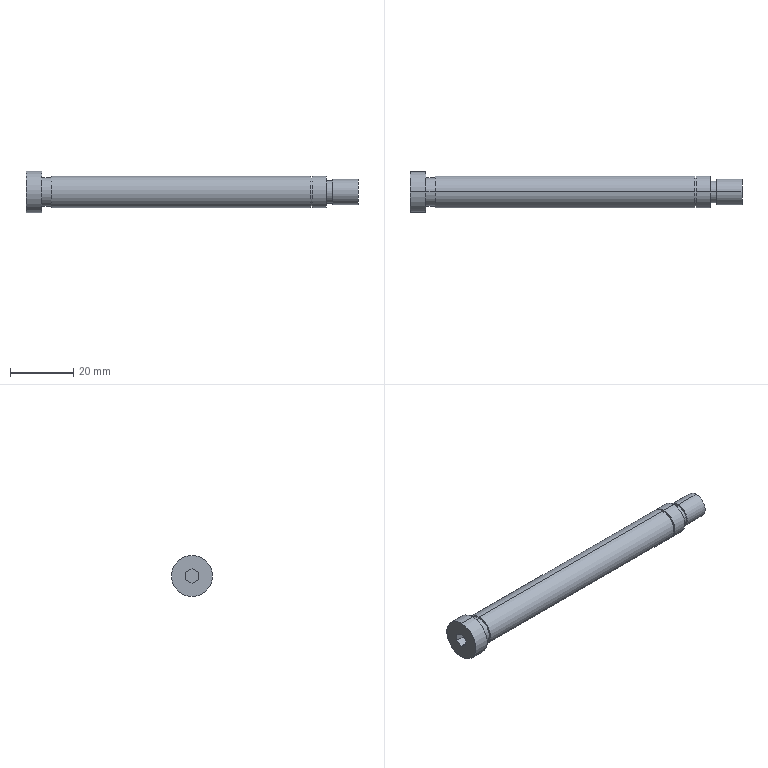Component | SolidWorks | ElectricalBoxAssembly2-1_M8-10-16-90GuidePinBolt-1 | 1 solid | 29 faces | box 105 x 13 x 13 mm | volume 8090 mm3 | plane 15 | cylinder 14 | commonest cylinder face diameters 10 x4 9 x4 7 x2 8 x2 13 x2
build123d program:
from build123d import *

# Parameters (mm, degrees)
SKETCH1_R           = 6.5
BOSS_EXTRUDE1_DEPTH = 5
SKETCH2_R           = 5
BOSS_EXTRUDE2_DEPTH = 90
SKETCH3_R           = 4
BOSS_EXTRUDE3_DEPTH = 10
SKETCH4_R           = 5
SKETCH4_R_2         = 4.5
CUT_EXTRUDE1_DEPTH  = 3
SKETCH5_R           = 4
SKETCH5_R_2         = 3.5
CUT_EXTRUDE2_DEPTH  = 2
CUT_EXTRUDE3_DEPTH  = 5
SKETCH7_W           = 0.5
SKETCH7_H           = 1


with BuildPart() as part:
    # Sketch1 → Boss-Extrude1 (new body)
    with BuildSketch(Plane.XY):
        Circle(SKETCH1_R)
    extrude(amount=-BOSS_EXTRUDE1_DEPTH)

    # Sketch2 → Boss-Extrude2 (add)
    with BuildSketch(Plane(origin=(0, 0, -5), x_dir=(-1, 0, 0), z_dir=(0, 0, -1))):
        with Locations(Location((0, 0, 0), (0, 0, 180))):
            Circle(SKETCH2_R)
    extrude(amount=BOSS_EXTRUDE2_DEPTH)

    # Sketch3 → Boss-Extrude3 (add)
    with BuildSketch(Plane(origin=(0, 0, -95), x_dir=(-1, 0, 0), z_dir=(0, 0, -1))):
        Circle(SKETCH3_R)
    extrude(amount=BOSS_EXTRUDE3_DEPTH)

    # Sketch4 → Cut-Extrude1 (cut)
    with BuildSketch(Plane(origin=(0, 0, -5), x_dir=(-1, 0, 0), z_dir=(0, 0, -1))):
        with Locations(Location((0, 0, 0), (0, 0, 180))):
            Circle(SKETCH4_R)
        Circle(SKETCH4_R_2, mode=Mode.SUBTRACT)
    extrude(amount=CUT_EXTRUDE1_DEPTH, mode=Mode.SUBTRACT)

    # Sketch5 → Cut-Extrude2 (cut)
    with BuildSketch(Plane(origin=(0, 0, -95), x_dir=(-1, 0, 0), z_dir=(0, 0, -1))):
        Circle(SKETCH5_R)
        Circle(SKETCH5_R_2, mode=Mode.SUBTRACT)
    extrude(amount=CUT_EXTRUDE2_DEPTH, mode=Mode.SUBTRACT)

    # Sketch6 → Cut-Extrude3 (cut)
    with BuildSketch(Plane.XY):
        Polygon((2.309, 0), (1.155, 2), (-1.155, 2), (-2.309, 0), (-1.155, -2), (1.155, -2), align=None)
    extrude(amount=-CUT_EXTRUDE3_DEPTH, mode=Mode.SUBTRACT)

    # Sketch7 → Cut-Revolve1 (revolve, cut)
    with BuildSketch(Plane(origin=(0, 0, 0), x_dir=(0, 0, -1), z_dir=(1, 0, 0)), mode=Mode.PRIVATE) as cut_revolve1_sk:
        with Locations((90.25, 5)):
            Rectangle(SKETCH7_W, SKETCH7_H)
    revolve(cut_revolve1_sk.sketch.rotate(Axis((0, 0, 0), (0, 0, -1)), 90), axis=Axis((0, 0, 0), (0, 0, -1)), mode=Mode.SUBTRACT)


solid = part.part

# Placed as in the assembly
solid = solid.moved(Location((640.968, 334.666, 1526.399), (0, -90, 0)))
STEP:
#1=COLOUR_RGB('',0.7922,0.8196,0.9333);
#2=FILL_AREA_STYLE_COLOUR('',#1);
#3=FILL_AREA_STYLE('',(#2));
#4=SURFACE_STYLE_FILL_AREA(#3);
#5=SURFACE_SIDE_STYLE('',(#4));
#6=SURFACE_STYLE_USAGE(.BOTH.,#5);
#7=PRESENTATION_STYLE_ASSIGNMENT((#6));
#8=CARTESIAN_POINT('',(28.975,13.176,60.291));
#9=VERTEX_POINT('',#8);
#10=CARTESIAN_POINT('',(28.975,13.176,59.898));
#11=VERTEX_POINT('',#10);
#12=CARTESIAN_POINT('',(28.975,13.176,60.094));
#13=DIRECTION('',(1.,0.,0.));
#14=DIRECTION('',(0.,0.,1.));
#15=AXIS2_PLACEMENT_3D('',#12,#13,#14);
#16=CIRCLE('',#15,0.1969);
#17=EDGE_CURVE('',#9,#11,#16,.T.);
#18=ORIENTED_EDGE('',*,*,#17,.F.);
#19=CARTESIAN_POINT('',(28.798,13.176,60.291));
#20=VERTEX_POINT('',#19);
#21=CARTESIAN_POINT('',(28.975,13.176,60.291));
#22=DIRECTION('',(-1.,-0.,-0.));
#23=VECTOR('',#22,39.37);
#24=LINE('',#21,#23);
#25=EDGE_CURVE('',#9,#20,#24,.T.);
#26=ORIENTED_EDGE('',*,*,#25,.T.);
#27=CARTESIAN_POINT('',(28.798,13.176,59.898));
#28=VERTEX_POINT('',#27);
#29=CARTESIAN_POINT('',(28.798,13.176,60.094));
#30=DIRECTION('',(-1.,-0.,-0.));
#31=DIRECTION('',(0.,1.,0.));
#32=AXIS2_PLACEMENT_3D('',#29,#30,#31);
#33=CIRCLE('',#32,0.1969);
#34=EDGE_CURVE('',#28,#20,#33,.T.);
#35=ORIENTED_EDGE('',*,*,#34,.F.);
#36=CARTESIAN_POINT('',(28.975,13.176,59.898));
#37=DIRECTION('',(-1.,-0.,-0.));
#38=VECTOR('',#37,39.37);
#39=LINE('',#36,#38);
#40=EDGE_CURVE('',#11,#28,#39,.T.);
#41=ORIENTED_EDGE('',*,*,#40,.F.);
#42=EDGE_LOOP('',(#18,#26,#35,#41));
#43=FACE_OUTER_BOUND('',#42,.T.);
#44=CARTESIAN_POINT('',(28.975,13.176,60.094));
#45=DIRECTION('',(-1.,-0.,-0.));
#46=DIRECTION('',(0.,0.,-1.));
#47=AXIS2_PLACEMENT_3D('',#44,#45,#46);
#48=CYLINDRICAL_SURFACE('',#47,0.1969);
#49=ADVANCED_FACE('',(#43),#48,.T.);
#50=CARTESIAN_POINT('',(29.054,13.176,60.232));
#51=VERTEX_POINT('',#50);
#52=CARTESIAN_POINT('',(29.054,13.176,59.957));
#53=VERTEX_POINT('',#52);
#54=CARTESIAN_POINT('',(29.054,13.176,60.094));
#55=DIRECTION('',(1.,0.,0.));
#56=DIRECTION('',(0.,0.,1.));
#57=AXIS2_PLACEMENT_3D('',#54,#55,#56);
#58=CIRCLE('',#57,0.1378);
#59=EDGE_CURVE('',#51,#53,#58,.T.);
#60=ORIENTED_EDGE('',*,*,#59,.F.);
#61=CARTESIAN_POINT('',(28.975,13.176,60.232));
#62=VERTEX_POINT('',#61);
#63=CARTESIAN_POINT('',(29.054,13.176,60.232));
#64=DIRECTION('',(-1.,-0.,-0.));
#65=VECTOR('',#64,39.37);
#66=LINE('',#63,#65);
#67=EDGE_CURVE('',#51,#62,#66,.T.);
#68=ORIENTED_EDGE('',*,*,#67,.T.);
#69=CARTESIAN_POINT('',(28.975,13.176,59.957));
#70=VERTEX_POINT('',#69);
#71=CARTESIAN_POINT('',(28.975,13.176,60.094));
#72=DIRECTION('',(1.,0.,0.));
#73=DIRECTION('',(0.,0.,1.));
#74=AXIS2_PLACEMENT_3D('',#71,#72,#73);
#75=CIRCLE('',#74,0.1378);
#76=EDGE_CURVE('',#62,#70,#75,.T.);
#77=ORIENTED_EDGE('',*,*,#76,.T.);
#78=CARTESIAN_POINT('',(29.054,13.176,59.957));
#79=DIRECTION('',(-1.,-0.,-0.));
#80=VECTOR('',#79,39.37);
#81=LINE('',#78,#80);
#82=EDGE_CURVE('',#53,#70,#81,.T.);
#83=ORIENTED_EDGE('',*,*,#82,.F.);
#84=EDGE_LOOP('',(#60,#68,#77,#83));
#85=FACE_OUTER_BOUND('',#84,.T.);
#86=CARTESIAN_POINT('',(29.054,13.176,60.094));
#87=DIRECTION('',(-1.,-0.,-0.));
#88=DIRECTION('',(0.,0.,-1.));
#89=AXIS2_PLACEMENT_3D('',#86,#87,#88);
#90=CYLINDRICAL_SURFACE('',#89,0.1378);
#91=ADVANCED_FACE('',(#85),#90,.T.);
#92=CARTESIAN_POINT('',(29.369,13.176,60.252));
#93=VERTEX_POINT('',#92);
#94=CARTESIAN_POINT('',(29.369,13.176,59.937));
#95=VERTEX_POINT('',#94);
#96=CARTESIAN_POINT('',(29.369,13.176,60.094));
#97=DIRECTION('',(1.,0.,0.));
#98=DIRECTION('',(0.,0.,1.));
#99=AXIS2_PLACEMENT_3D('',#96,#97,#98);
#100=CIRCLE('',#99,0.1575);
#101=EDGE_CURVE('',#93,#95,#100,.T.);
#102=ORIENTED_EDGE('',*,*,#101,.F.);
#103=CARTESIAN_POINT('',(29.054,13.176,60.252));
#104=VERTEX_POINT('',#103);
#105=CARTESIAN_POINT('',(29.369,13.176,60.252));
#106=DIRECTION('',(-1.,-0.,-0.));
#107=VECTOR('',#106,39.37);
#108=LINE('',#105,#107);
#109=EDGE_CURVE('',#93,#104,#108,.T.);
#110=ORIENTED_EDGE('',*,*,#109,.T.);
#111=CARTESIAN_POINT('',(29.054,13.176,59.937));
#112=VERTEX_POINT('',#111);
#113=CARTESIAN_POINT('',(29.054,13.176,60.094));
#114=DIRECTION('',(1.,0.,0.));
#115=DIRECTION('',(0.,0.,1.));
#116=AXIS2_PLACEMENT_3D('',#113,#114,#115);
#117=CIRCLE('',#116,0.1575);
#118=EDGE_CURVE('',#104,#112,#117,.T.);
#119=ORIENTED_EDGE('',*,*,#118,.T.);
#120=CARTESIAN_POINT('',(29.369,13.176,59.937));
#121=DIRECTION('',(-1.,-0.,-0.));
#122=VECTOR('',#121,39.37);
#123=LINE('',#120,#122);
#124=EDGE_CURVE('',#95,#112,#123,.T.);
#125=ORIENTED_EDGE('',*,*,#124,.F.);
#126=EDGE_LOOP('',(#102,#110,#119,#125));
#127=FACE_OUTER_BOUND('',#126,.T.);
#128=CARTESIAN_POINT('',(29.369,13.176,60.094));
#129=DIRECTION('',(-1.,-0.,-0.));
#130=DIRECTION('',(0.,0.,-1.));
#131=AXIS2_PLACEMENT_3D('',#128,#129,#130);
#132=CYLINDRICAL_SURFACE('',#131,0.1575);
#133=ADVANCED_FACE('',(#127),#132,.T.);
#134=CARTESIAN_POINT('',(28.798,13.353,60.094));
#135=VERTEX_POINT('',#134);
#136=CARTESIAN_POINT('',(28.798,12.999,60.094));
#137=VERTEX_POINT('',#136);
#138=CARTESIAN_POINT('',(28.798,13.176,60.094));
#139=DIRECTION('',(-1.,-0.,-0.));
#140=DIRECTION('',(0.,1.,0.));
#141=AXIS2_PLACEMENT_3D('',#138,#139,#140);
#142=CIRCLE('',#141,0.1772);
#143=EDGE_CURVE('',#135,#137,#142,.T.);
#144=ORIENTED_EDGE('',*,*,#143,.T.);
#145=CARTESIAN_POINT('',(28.778,12.999,60.094));
#146=VERTEX_POINT('',#145);
#147=CARTESIAN_POINT('',(25.235,12.999,60.094));
#148=DIRECTION('',(-1.,-0.,-0.));
#149=VECTOR('',#148,39.37);
#150=LINE('',#147,#149);
#151=EDGE_CURVE('',#137,#146,#150,.T.);
#152=ORIENTED_EDGE('',*,*,#151,.T.);
#153=CARTESIAN_POINT('',(28.778,13.353,60.094));
#154=VERTEX_POINT('',#153);
#155=CARTESIAN_POINT('',(28.778,13.176,60.094));
#156=DIRECTION('',(-1.,-0.,-0.));
#157=DIRECTION('',(0.,1.,0.));
#158=AXIS2_PLACEMENT_3D('',#155,#156,#157);
#159=CIRCLE('',#158,0.1772);
#160=EDGE_CURVE('',#154,#146,#159,.T.);
#161=ORIENTED_EDGE('',*,*,#160,.F.);
#162=CARTESIAN_POINT('',(25.235,13.353,60.094));
#163=DIRECTION('',(-1.,-0.,-0.));
#164=VECTOR('',#163,39.37);
#165=LINE('',#162,#164);
#166=EDGE_CURVE('',#135,#154,#165,.T.);
#167=ORIENTED_EDGE('',*,*,#166,.F.);
#168=EDGE_LOOP('',(#144,#152,#161,#167));
#169=FACE_OUTER_BOUND('',#168,.T.);
#170=CARTESIAN_POINT('',(25.235,13.176,60.094));
#171=DIRECTION('',(-1.,-0.,-0.));
#172=DIRECTION('',(0.,1.,0.));
#173=AXIS2_PLACEMENT_3D('',#170,#171,#172);
#174=CYLINDRICAL_SURFACE('',#173,0.1772);
#175=ADVANCED_FACE('',(#169),#174,.T.);
#176=CARTESIAN_POINT('',(25.432,13.176,59.839));
#177=VERTEX_POINT('',#176);
#178=CARTESIAN_POINT('',(25.432,13.176,60.35));
#179=VERTEX_POINT('',#178);
#180=CARTESIAN_POINT('',(25.432,13.176,60.094));
#181=DIRECTION('',(-1.,-0.,-0.));
#182=DIRECTION('',(0.,0.,-1.));
#183=AXIS2_PLACEMENT_3D('',#180,#181,#182);
#184=CIRCLE('',#183,0.2559);
#185=EDGE_CURVE('',#177,#179,#184,.T.);
#186=ORIENTED_EDGE('',*,*,#185,.T.);
#187=CARTESIAN_POINT('',(25.235,13.176,60.35));
#188=VERTEX_POINT('',#187);
#189=CARTESIAN_POINT('',(25.432,13.176,60.35));
#190=DIRECTION('',(-1.,-0.,-0.));
#191=VECTOR('',#190,39.37);
#192=LINE('',#189,#191);
#193=EDGE_CURVE('',#179,#188,#192,.T.);
#194=ORIENTED_EDGE('',*,*,#193,.T.);
#195=CARTESIAN_POINT('',(25.235,13.176,59.839));
#196=VERTEX_POINT('',#195);
#197=CARTESIAN_POINT('',(25.235,13.176,60.094));
#198=DIRECTION('',(-1.,-0.,-0.));
#199=DIRECTION('',(0.,0.,-1.));
#200=AXIS2_PLACEMENT_3D('',#197,#198,#199);
#201=CIRCLE('',#200,0.2559);
#202=EDGE_CURVE('',#196,#188,#201,.T.);
#203=ORIENTED_EDGE('',*,*,#202,.F.);
#204=CARTESIAN_POINT('',(25.432,13.176,59.839));
#205=DIRECTION('',(-1.,-0.,-0.));
#206=VECTOR('',#205,39.37);
#207=LINE('',#204,#206);
#208=EDGE_CURVE('',#177,#196,#207,.T.);
#209=ORIENTED_EDGE('',*,*,#208,.F.);
#210=EDGE_LOOP('',(#186,#194,#203,#209));
#211=FACE_OUTER_BOUND('',#210,.T.);
#212=CARTESIAN_POINT('',(25.432,13.176,60.094));
#213=DIRECTION('',(-1.,-0.,-0.));
#214=DIRECTION('',(0.,0.,-1.));
#215=AXIS2_PLACEMENT_3D('',#212,#213,#214);
#216=CYLINDRICAL_SURFACE('',#215,0.2559);
#217=ADVANCED_FACE('',(#211),#216,.T.);
#218=CARTESIAN_POINT('',(25.55,13.176,60.272));
#219=VERTEX_POINT('',#218);
#220=CARTESIAN_POINT('',(25.55,13.176,59.917));
#221=VERTEX_POINT('',#220);
#222=CARTESIAN_POINT('',(25.55,13.176,60.094));
#223=DIRECTION('',(1.,0.,0.));
#224=DIRECTION('',(0.,0.,1.));
#225=AXIS2_PLACEMENT_3D('',#222,#223,#224);
#226=CIRCLE('',#225,0.1772);
#227=EDGE_CURVE('',#219,#221,#226,.T.);
#228=ORIENTED_EDGE('',*,*,#227,.F.);
#229=CARTESIAN_POINT('',(25.432,13.176,60.272));
#230=VERTEX_POINT('',#229);
#231=CARTESIAN_POINT('',(25.55,13.176,60.272));
#232=DIRECTION('',(-1.,-0.,-0.));
#233=VECTOR('',#232,39.37);
#234=LINE('',#231,#233);
#235=EDGE_CURVE('',#219,#230,#234,.T.);
#236=ORIENTED_EDGE('',*,*,#235,.T.);
#237=CARTESIAN_POINT('',(25.432,13.176,59.917));
#238=VERTEX_POINT('',#237);
#239=CARTESIAN_POINT('',(25.432,13.176,60.094));
#240=DIRECTION('',(1.,0.,0.));
#241=DIRECTION('',(0.,0.,1.));
#242=AXIS2_PLACEMENT_3D('',#239,#240,#241);
#243=CIRCLE('',#242,0.1772);
#244=EDGE_CURVE('',#230,#238,#243,.T.);
#245=ORIENTED_EDGE('',*,*,#244,.T.);
#246=CARTESIAN_POINT('',(25.55,13.176,59.917));
#247=DIRECTION('',(-1.,-0.,-0.));
#248=VECTOR('',#247,39.37);
#249=LINE('',#246,#248);
#250=EDGE_CURVE('',#221,#238,#249,.T.);
#251=ORIENTED_EDGE('',*,*,#250,.F.);
#252=EDGE_LOOP('',(#228,#236,#245,#251));
#253=FACE_OUTER_BOUND('',#252,.T.);
#254=CARTESIAN_POINT('',(25.55,13.176,60.094));
#255=DIRECTION('',(-1.,-0.,-0.));
#256=DIRECTION('',(0.,0.,-1.));
#257=AXIS2_PLACEMENT_3D('',#254,#255,#256);
#258=CYLINDRICAL_SURFACE('',#257,0.1772);
#259=ADVANCED_FACE('',(#253),#258,.T.);
#260=CARTESIAN_POINT('',(28.778,13.176,60.291));
#261=VERTEX_POINT('',#260);
#262=CARTESIAN_POINT('',(28.778,13.176,59.898));
#263=VERTEX_POINT('',#262);
#264=CARTESIAN_POINT('',(28.778,13.176,60.094));
#265=DIRECTION('',(1.,0.,0.));
#266=DIRECTION('',(0.,-1.,0.));
#267=AXIS2_PLACEMENT_3D('',#264,#265,#266);
#268=CIRCLE('',#267,0.1969);
#269=EDGE_CURVE('',#261,#263,#268,.T.);
#270=ORIENTED_EDGE('',*,*,#269,.F.);
#271=CARTESIAN_POINT('',(25.55,13.176,60.291));
#272=VERTEX_POINT('',#271);
#273=CARTESIAN_POINT('',(28.975,13.176,60.291));
#274=DIRECTION('',(-1.,-0.,-0.));
#275=VECTOR('',#274,39.37);
#276=LINE('',#273,#275);
#277=EDGE_CURVE('',#261,#272,#276,.T.);
#278=ORIENTED_EDGE('',*,*,#277,.T.);
#279=CARTESIAN_POINT('',(25.55,13.176,59.898));
#280=VERTEX_POINT('',#279);
#281=CARTESIAN_POINT('',(25.55,13.176,60.094));
#282=DIRECTION('',(1.,0.,0.));
#283=DIRECTION('',(0.,0.,1.));
#284=AXIS2_PLACEMENT_3D('',#281,#282,#283);
#285=CIRCLE('',#284,0.1969);
#286=EDGE_CURVE('',#272,#280,#285,.T.);
#287=ORIENTED_EDGE('',*,*,#286,.T.);
#288=CARTESIAN_POINT('',(28.975,13.176,59.898));
#289=DIRECTION('',(-1.,-0.,-0.));
#290=VECTOR('',#289,39.37);
#291=LINE('',#288,#290);
#292=EDGE_CURVE('',#263,#280,#291,.T.);
#293=ORIENTED_EDGE('',*,*,#292,.F.);
#294=EDGE_LOOP('',(#270,#278,#287,#293));
#295=FACE_OUTER_BOUND('',#294,.T.);
#296=CARTESIAN_POINT('',(28.975,13.176,60.094));
#297=DIRECTION('',(-1.,-0.,-0.));
#298=DIRECTION('',(0.,0.,-1.));
#299=AXIS2_PLACEMENT_3D('',#296,#297,#298);
#300=CYLINDRICAL_SURFACE('',#299,0.1969);
#301=ADVANCED_FACE('',(#295),#300,.T.);
#302=ORIENTED_EDGE('',*,*,#277,.F.);
#303=CARTESIAN_POINT('',(28.778,13.176,60.094));
#304=DIRECTION('',(1.,0.,0.));
#305=DIRECTION('',(0.,-1.,0.));
#306=AXIS2_PLACEMENT_3D('',#303,#304,#305);
#307=CIRCLE('',#306,0.1969);
#308=EDGE_CURVE('',#263,#261,#307,.T.);
#309=ORIENTED_EDGE('',*,*,#308,.F.);
#310=ORIENTED_EDGE('',*,*,#292,.T.);
#311=CARTESIAN_POINT('',(25.55,13.176,60.094));
#312=DIRECTION('',(1.,0.,0.));
#313=DIRECTION('',(0.,0.,1.));
#314=AXIS2_PLACEMENT_3D('',#311,#312,#313);
#315=CIRCLE('',#314,0.1969);
#316=EDGE_CURVE('',#280,#272,#315,.T.);
#317=ORIENTED_EDGE('',*,*,#316,.T.);
#318=EDGE_LOOP('',(#302,#309,#310,#317));
#319=FACE_OUTER_BOUND('',#318,.T.);
#320=CARTESIAN_POINT('',(28.975,13.176,60.094));
#321=DIRECTION('',(-1.,-0.,-0.));
#322=DIRECTION('',(0.,0.,-1.));
#323=AXIS2_PLACEMENT_3D('',#320,#321,#322);
#324=CYLINDRICAL_SURFACE('',#323,0.1969);
#325=ADVANCED_FACE('',(#319),#324,.T.);
#326=ORIENTED_EDGE('',*,*,#316,.F.);
#327=ORIENTED_EDGE('',*,*,#286,.F.);
#328=EDGE_LOOP('',(#326,#327));
#329=FACE_OUTER_BOUND('',#328,.T.);
#330=CARTESIAN_POINT('',(25.55,13.176,60.094));
#331=DIRECTION('',(1.,0.,0.));
#332=DIRECTION('',(0.,0.,1.));
#333=AXIS2_PLACEMENT_3D('',#330,#331,#332);
#334=CIRCLE('',#333,0.1772);
#335=EDGE_CURVE('',#221,#219,#334,.T.);
#336=ORIENTED_EDGE('',*,*,#335,.T.);
#337=ORIENTED_EDGE('',*,*,#227,.T.);
#338=EDGE_LOOP('',(#336,#337));
#339=FACE_BOUND('',#338,.T.);
#340=CARTESIAN_POINT('',(25.55,13.176,60.094));
#341=DIRECTION('',(1.,0.,0.));
#342=DIRECTION('',(-0.,0.,1.));
#343=AXIS2_PLACEMENT_3D('',#340,#341,#342);
#344=PLANE('',#343);
#345=ADVANCED_FACE('',(#329,#339),#344,.F.);
#346=ORIENTED_EDGE('',*,*,#235,.F.);
#347=ORIENTED_EDGE('',*,*,#335,.F.);
#348=ORIENTED_EDGE('',*,*,#250,.T.);
#349=CARTESIAN_POINT('',(25.432,13.176,60.094));
#350=DIRECTION('',(1.,0.,0.));
#351=DIRECTION('',(0.,0.,1.));
#352=AXIS2_PLACEMENT_3D('',#349,#350,#351);
#353=CIRCLE('',#352,0.1772);
#354=EDGE_CURVE('',#238,#230,#353,.T.);
#355=ORIENTED_EDGE('',*,*,#354,.T.);
#356=EDGE_LOOP('',(#346,#347,#348,#355));
#357=FACE_OUTER_BOUND('',#356,.T.);
#358=CARTESIAN_POINT('',(25.55,13.176,60.094));
#359=DIRECTION('',(-1.,-0.,-0.));
#360=DIRECTION('',(0.,0.,-1.));
#361=AXIS2_PLACEMENT_3D('',#358,#359,#360);
#362=CYLINDRICAL_SURFACE('',#361,0.1772);
#363=ADVANCED_FACE('',(#357),#362,.T.);
#364=CARTESIAN_POINT('',(25.235,13.255,60.049));
#365=VERTEX_POINT('',#364);
#366=CARTESIAN_POINT('',(25.235,13.176,60.004));
#367=VERTEX_POINT('',#366);
#368=CARTESIAN_POINT('',(25.235,13.255,60.049));
#369=DIRECTION('',(0.,-0.866,-0.5));
#370=VECTOR('',#369,39.37);
#371=LINE('',#368,#370);
#372=EDGE_CURVE('',#365,#367,#371,.T.);
#373=ORIENTED_EDGE('',*,*,#372,.F.);
#374=CARTESIAN_POINT('',(25.235,13.255,60.14));
#375=VERTEX_POINT('',#374);
#376=CARTESIAN_POINT('',(25.235,13.255,60.14));
#377=DIRECTION('',(0.,0.,-1.));
#378=VECTOR('',#377,39.37);
#379=LINE('',#376,#378);
#380=EDGE_CURVE('',#375,#365,#379,.T.);
#381=ORIENTED_EDGE('',*,*,#380,.F.);
#382=CARTESIAN_POINT('',(25.235,13.176,60.185));
#383=VERTEX_POINT('',#382);
#384=CARTESIAN_POINT('',(25.235,13.176,60.185));
#385=DIRECTION('',(0.,0.866,-0.5));
#386=VECTOR('',#385,39.37);
#387=LINE('',#384,#386);
#388=EDGE_CURVE('',#383,#375,#387,.T.);
#389=ORIENTED_EDGE('',*,*,#388,.F.);
#390=CARTESIAN_POINT('',(25.235,13.097,60.14));
#391=VERTEX_POINT('',#390);
#392=CARTESIAN_POINT('',(25.235,13.097,60.14));
#393=DIRECTION('',(-0.,0.866,0.5));
#394=VECTOR('',#393,39.37);
#395=LINE('',#392,#394);
#396=EDGE_CURVE('',#391,#383,#395,.T.);
#397=ORIENTED_EDGE('',*,*,#396,.F.);
#398=CARTESIAN_POINT('',(25.235,13.097,60.049));
#399=VERTEX_POINT('',#398);
#400=CARTESIAN_POINT('',(25.235,13.097,60.049));
#401=DIRECTION('',(-0.,0.,1.));
#402=VECTOR('',#401,39.37);
#403=LINE('',#400,#402);
#404=EDGE_CURVE('',#399,#391,#403,.T.);
#405=ORIENTED_EDGE('',*,*,#404,.F.);
#406=CARTESIAN_POINT('',(25.235,13.176,60.004));
#407=DIRECTION('',(-0.,-0.866,0.5));
#408=VECTOR('',#407,39.37);
#409=LINE('',#406,#408);
#410=EDGE_CURVE('',#367,#399,#409,.T.);
#411=ORIENTED_EDGE('',*,*,#410,.F.);
#412=EDGE_LOOP('',(#373,#381,#389,#397,#405,#411));
#413=FACE_BOUND('',#412,.T.);
#414=ORIENTED_EDGE('',*,*,#202,.T.);
#415=CARTESIAN_POINT('',(25.235,13.176,60.094));
#416=DIRECTION('',(-1.,-0.,-0.));
#417=DIRECTION('',(0.,0.,-1.));
#418=AXIS2_PLACEMENT_3D('',#415,#416,#417);
#419=CIRCLE('',#418,0.2559);
#420=EDGE_CURVE('',#188,#196,#419,.T.);
#421=ORIENTED_EDGE('',*,*,#420,.T.);
#422=EDGE_LOOP('',(#414,#421));
#423=FACE_OUTER_BOUND('',#422,.T.);
#424=CARTESIAN_POINT('',(25.235,13.176,60.094));
#425=DIRECTION('',(-1.,-0.,-0.));
#426=DIRECTION('',(0.,-0.,-1.));
#427=AXIS2_PLACEMENT_3D('',#424,#425,#426);
#428=PLANE('',#427);
#429=ADVANCED_FACE('',(#413,#423),#428,.T.);
#430=ORIENTED_EDGE('',*,*,#193,.F.);
#431=CARTESIAN_POINT('',(25.432,13.176,60.094));
#432=DIRECTION('',(-1.,-0.,-0.));
#433=DIRECTION('',(0.,0.,-1.));
#434=AXIS2_PLACEMENT_3D('',#431,#432,#433);
#435=CIRCLE('',#434,0.2559);
#436=EDGE_CURVE('',#179,#177,#435,.T.);
#437=ORIENTED_EDGE('',*,*,#436,.T.);
#438=ORIENTED_EDGE('',*,*,#208,.T.);
#439=ORIENTED_EDGE('',*,*,#420,.F.);
#440=EDGE_LOOP('',(#430,#437,#438,#439));
#441=FACE_OUTER_BOUND('',#440,.T.);
#442=CARTESIAN_POINT('',(25.432,13.176,60.094));
#443=DIRECTION('',(-1.,-0.,-0.));
#444=DIRECTION('',(0.,0.,-1.));
#445=AXIS2_PLACEMENT_3D('',#442,#443,#444);
#446=CYLINDRICAL_SURFACE('',#445,0.2559);
#447=ADVANCED_FACE('',(#441),#446,.T.);
#448=ORIENTED_EDGE('',*,*,#185,.F.);
#449=ORIENTED_EDGE('',*,*,#436,.F.);
#450=EDGE_LOOP('',(#448,#449));
#451=FACE_OUTER_BOUND('',#450,.T.);
#452=ORIENTED_EDGE('',*,*,#354,.F.);
#453=ORIENTED_EDGE('',*,*,#244,.F.);
#454=EDGE_LOOP('',(#452,#453));
#455=FACE_BOUND('',#454,.T.);
#456=CARTESIAN_POINT('',(25.432,13.176,60.094));
#457=DIRECTION('',(-1.,-0.,-0.));
#458=DIRECTION('',(0.,-0.,-1.));
#459=AXIS2_PLACEMENT_3D('',#456,#457,#458);
#460=PLANE('',#459);
#461=ADVANCED_FACE('',(#451,#455),#460,.F.);
#462=ORIENTED_EDGE('',*,*,#372,.T.);
#463=CARTESIAN_POINT('',(25.432,13.176,60.004));
#464=VERTEX_POINT('',#463);
#465=CARTESIAN_POINT('',(25.432,13.176,60.004));
#466=DIRECTION('',(-1.,-0.,-0.));
#467=VECTOR('',#466,39.37);
#468=LINE('',#465,#467);
#469=EDGE_CURVE('',#464,#367,#468,.T.);
#470=ORIENTED_EDGE('',*,*,#469,.F.);
#471=CARTESIAN_POINT('',(25.432,13.255,60.049));
#472=VERTEX_POINT('',#471);
#473=CARTESIAN_POINT('',(25.432,13.255,60.049));
#474=DIRECTION('',(0.,-0.866,-0.5));
#475=VECTOR('',#474,39.37);
#476=LINE('',#473,#475);
#477=EDGE_CURVE('',#472,#464,#476,.T.);
#478=ORIENTED_EDGE('',*,*,#477,.F.);
#479=CARTESIAN_POINT('',(25.432,13.255,60.049));
#480=DIRECTION('',(-1.,-0.,-0.));
#481=VECTOR('',#480,39.37);
#482=LINE('',#479,#481);
#483=EDGE_CURVE('',#472,#365,#482,.T.);
#484=ORIENTED_EDGE('',*,*,#483,.T.);
#485=EDGE_LOOP('',(#462,#470,#478,#484));
#486=FACE_OUTER_BOUND('',#485,.T.);
#487=CARTESIAN_POINT('',(25.432,13.255,60.049));
#488=DIRECTION('',(0.,0.5,-0.866));
#489=DIRECTION('',(0.,-0.866,-0.5));
#490=AXIS2_PLACEMENT_3D('',#487,#488,#489);
#491=PLANE('',#490);
#492=ADVANCED_FACE('',(#486),#491,.F.);
#493=ORIENTED_EDGE('',*,*,#380,.T.);
#494=ORIENTED_EDGE('',*,*,#483,.F.);
#495=CARTESIAN_POINT('',(25.432,13.255,60.14));
#496=VERTEX_POINT('',#495);
#497=CARTESIAN_POINT('',(25.432,13.255,60.14));
#498=DIRECTION('',(0.,0.,-1.));
#499=VECTOR('',#498,39.37);
#500=LINE('',#497,#499);
#501=EDGE_CURVE('',#496,#472,#500,.T.);
#502=ORIENTED_EDGE('',*,*,#501,.F.);
#503=CARTESIAN_POINT('',(25.432,13.255,60.14));
#504=DIRECTION('',(-1.,-0.,-0.));
#505=VECTOR('',#504,39.37);
#506=LINE('',#503,#505);
#507=EDGE_CURVE('',#496,#375,#506,.T.);
#508=ORIENTED_EDGE('',*,*,#507,.T.);
#509=EDGE_LOOP('',(#493,#494,#502,#508));
#510=FACE_OUTER_BOUND('',#509,.T.);
#511=CARTESIAN_POINT('',(25.432,13.255,60.14));
#512=DIRECTION('',(-0.,1.,0.));
#513=DIRECTION('',(0.,0.,-1.));
#514=AXIS2_PLACEMENT_3D('',#511,#512,#513);
#515=PLANE('',#514);
#516=ADVANCED_FACE('',(#510),#515,.F.);
#517=ORIENTED_EDGE('',*,*,#388,.T.);
#518=ORIENTED_EDGE('',*,*,#507,.F.);
#519=CARTESIAN_POINT('',(25.432,13.176,60.185));
#520=VERTEX_POINT('',#519);
#521=CARTESIAN_POINT('',(25.432,13.176,60.185));
#522=DIRECTION('',(0.,0.866,-0.5));
#523=VECTOR('',#522,39.37);
#524=LINE('',#521,#523);
#525=EDGE_CURVE('',#520,#496,#524,.T.);
#526=ORIENTED_EDGE('',*,*,#525,.F.);
#527=CARTESIAN_POINT('',(25.432,13.176,60.185));
#528=DIRECTION('',(-1.,-0.,-0.));
#529=VECTOR('',#528,39.37);
#530=LINE('',#527,#529);
#531=EDGE_CURVE('',#520,#383,#530,.T.);
#532=ORIENTED_EDGE('',*,*,#531,.T.);
#533=EDGE_LOOP('',(#517,#518,#526,#532));
#534=FACE_OUTER_BOUND('',#533,.T.);
#535=CARTESIAN_POINT('',(25.432,13.176,60.185));
#536=DIRECTION('',(-0.,0.5,0.866));
#537=DIRECTION('',(0.,0.866,-0.5));
#538=AXIS2_PLACEMENT_3D('',#535,#536,#537);
#539=PLANE('',#538);
#540=ADVANCED_FACE('',(#534),#539,.F.);
#541=ORIENTED_EDGE('',*,*,#396,.T.);
#542=ORIENTED_EDGE('',*,*,#531,.F.);
#543=CARTESIAN_POINT('',(25.432,13.097,60.14));
#544=VERTEX_POINT('',#543);
#545=CARTESIAN_POINT('',(25.432,13.097,60.14));
#546=DIRECTION('',(-0.,0.866,0.5));
#547=VECTOR('',#546,39.37);
#548=LINE('',#545,#547);
#549=EDGE_CURVE('',#544,#520,#548,.T.);
#550=ORIENTED_EDGE('',*,*,#549,.F.);
#551=CARTESIAN_POINT('',(25.432,13.097,60.14));
#552=DIRECTION('',(-1.,-0.,-0.));
#553=VECTOR('',#552,39.37);
#554=LINE('',#551,#553);
#555=EDGE_CURVE('',#544,#391,#554,.T.);
#556=ORIENTED_EDGE('',*,*,#555,.T.);
#557=EDGE_LOOP('',(#541,#542,#550,#556));
#558=FACE_OUTER_BOUND('',#557,.T.);
#559=CARTESIAN_POINT('',(25.432,13.097,60.14));
#560=DIRECTION('',(-0.,-0.5,0.866));
#561=DIRECTION('',(-0.,0.866,0.5));
#562=AXIS2_PLACEMENT_3D('',#559,#560,#561);
#563=PLANE('',#562);
#564=ADVANCED_FACE('',(#558),#563,.F.);
#565=ORIENTED_EDGE('',*,*,#404,.T.);
#566=ORIENTED_EDGE('',*,*,#555,.F.);
#567=CARTESIAN_POINT('',(25.432,13.097,60.049));
#568=VERTEX_POINT('',#567);
#569=CARTESIAN_POINT('',(25.432,13.097,60.049));
#570=DIRECTION('',(-0.,0.,1.));
#571=VECTOR('',#570,39.37);
#572=LINE('',#569,#571);
#573=EDGE_CURVE('',#568,#544,#572,.T.);
#574=ORIENTED_EDGE('',*,*,#573,.F.);
#575=CARTESIAN_POINT('',(25.432,13.097,60.049));
#576=DIRECTION('',(-1.,-0.,-0.));
#577=VECTOR('',#576,39.37);
#578=LINE('',#575,#577);
#579=EDGE_CURVE('',#568,#399,#578,.T.);
#580=ORIENTED_EDGE('',*,*,#579,.T.);
#581=EDGE_LOOP('',(#565,#566,#574,#580));
#582=FACE_OUTER_BOUND('',#581,.T.);
#583=CARTESIAN_POINT('',(25.432,13.097,60.049));
#584=DIRECTION('',(0.,-1.,-0.));
#585=DIRECTION('',(-1.,-0.,-0.));
#586=AXIS2_PLACEMENT_3D('',#583,#584,#585);
#587=PLANE('',#586);
#588=ADVANCED_FACE('',(#582),#587,.F.);
#589=ORIENTED_EDGE('',*,*,#410,.T.);
#590=ORIENTED_EDGE('',*,*,#579,.F.);
#591=CARTESIAN_POINT('',(25.432,13.176,60.004));
#592=DIRECTION('',(-0.,-0.866,0.5));
#593=VECTOR('',#592,39.37);
#594=LINE('',#591,#593);
#595=EDGE_CURVE('',#464,#568,#594,.T.);
#596=ORIENTED_EDGE('',*,*,#595,.F.);
#597=ORIENTED_EDGE('',*,*,#469,.T.);
#598=EDGE_LOOP('',(#589,#590,#596,#597));
#599=FACE_OUTER_BOUND('',#598,.T.);
#600=CARTESIAN_POINT('',(25.432,13.176,60.004));
#601=DIRECTION('',(0.,-0.5,-0.866));
#602=DIRECTION('',(-0.,-0.866,0.5));
#603=AXIS2_PLACEMENT_3D('',#600,#601,#602);
#604=PLANE('',#603);
#605=ADVANCED_FACE('',(#599),#604,.F.);
#606=ORIENTED_EDGE('',*,*,#477,.T.);
#607=ORIENTED_EDGE('',*,*,#595,.T.);
#608=ORIENTED_EDGE('',*,*,#573,.T.);
#609=ORIENTED_EDGE('',*,*,#549,.T.);
#610=ORIENTED_EDGE('',*,*,#525,.T.);
#611=ORIENTED_EDGE('',*,*,#501,.T.);
#612=EDGE_LOOP('',(#606,#607,#608,#609,#610,#611));
#613=FACE_OUTER_BOUND('',#612,.T.);
#614=CARTESIAN_POINT('',(25.432,13.176,60.094));
#615=DIRECTION('',(-1.,-0.,-0.));
#616=DIRECTION('',(0.,-0.,-1.));
#617=AXIS2_PLACEMENT_3D('',#614,#615,#616);
#618=PLANE('',#617);
#619=ADVANCED_FACE('',(#613),#618,.T.);
#620=ORIENTED_EDGE('',*,*,#143,.F.);
#621=CARTESIAN_POINT('',(28.798,13.176,60.094));
#622=DIRECTION('',(-1.,-0.,-0.));
#623=DIRECTION('',(0.,1.,0.));
#624=AXIS2_PLACEMENT_3D('',#621,#622,#623);
#625=CIRCLE('',#624,0.1772);
#626=EDGE_CURVE('',#137,#135,#625,.T.);
#627=ORIENTED_EDGE('',*,*,#626,.F.);
#628=EDGE_LOOP('',(#620,#627));
#629=FACE_BOUND('',#628,.T.);
#630=ORIENTED_EDGE('',*,*,#34,.T.);
#631=CARTESIAN_POINT('',(28.798,13.176,60.094));
#632=DIRECTION('',(-1.,-0.,-0.));
#633=DIRECTION('',(0.,1.,0.));
#634=AXIS2_PLACEMENT_3D('',#631,#632,#633);
#635=CIRCLE('',#634,0.1969);
#636=EDGE_CURVE('',#20,#28,#635,.T.);
#637=ORIENTED_EDGE('',*,*,#636,.T.);
#638=EDGE_LOOP('',(#630,#637));
#639=FACE_OUTER_BOUND('',#638,.T.);
#640=CARTESIAN_POINT('',(28.798,12.959,60.094));
#641=DIRECTION('',(-1.,-0.,-0.));
#642=DIRECTION('',(-0.,1.,0.));
#643=AXIS2_PLACEMENT_3D('',#640,#641,#642);
#644=PLANE('',#643);
#645=ADVANCED_FACE('',(#629,#639),#644,.T.);
#646=ORIENTED_EDGE('',*,*,#160,.T.);
#647=CARTESIAN_POINT('',(28.778,13.176,60.094));
#648=DIRECTION('',(-1.,-0.,-0.));
#649=DIRECTION('',(0.,1.,0.));
#650=AXIS2_PLACEMENT_3D('',#647,#648,#649);
#651=CIRCLE('',#650,0.1772);
#652=EDGE_CURVE('',#146,#154,#651,.T.);
#653=ORIENTED_EDGE('',*,*,#652,.T.);
#654=EDGE_LOOP('',(#646,#653));
#655=FACE_BOUND('',#654,.T.);
#656=ORIENTED_EDGE('',*,*,#308,.T.);
#657=ORIENTED_EDGE('',*,*,#269,.T.);
#658=EDGE_LOOP('',(#656,#657));
#659=FACE_OUTER_BOUND('',#658,.T.);
#660=CARTESIAN_POINT('',(28.778,12.959,60.094));
#661=DIRECTION('',(1.,0.,0.));
#662=DIRECTION('',(0.,-1.,-0.));
#663=AXIS2_PLACEMENT_3D('',#660,#661,#662);
#664=PLANE('',#663);
#665=ADVANCED_FACE('',(#655,#659),#664,.T.);
#666=ORIENTED_EDGE('',*,*,#151,.F.);
#667=ORIENTED_EDGE('',*,*,#626,.T.);
#668=ORIENTED_EDGE('',*,*,#166,.T.);
#669=ORIENTED_EDGE('',*,*,#652,.F.);
#670=EDGE_LOOP('',(#666,#667,#668,#669));
#671=FACE_OUTER_BOUND('',#670,.T.);
#672=CARTESIAN_POINT('',(25.235,13.176,60.094));
#673=DIRECTION('',(-1.,-0.,-0.));
#674=DIRECTION('',(0.,1.,0.));
#675=AXIS2_PLACEMENT_3D('',#672,#673,#674);
#676=CYLINDRICAL_SURFACE('',#675,0.1772);
#677=ADVANCED_FACE('',(#671),#676,.T.);
#678=CARTESIAN_POINT('',(29.369,13.176,60.094));
#679=DIRECTION('',(1.,0.,0.));
#680=DIRECTION('',(0.,0.,1.));
#681=AXIS2_PLACEMENT_3D('',#678,#679,#680);
#682=CIRCLE('',#681,0.1575);
#683=EDGE_CURVE('',#95,#93,#682,.T.);
#684=ORIENTED_EDGE('',*,*,#683,.T.);
#685=ORIENTED_EDGE('',*,*,#101,.T.);
#686=EDGE_LOOP('',(#684,#685));
#687=FACE_OUTER_BOUND('',#686,.T.);
#688=CARTESIAN_POINT('',(29.369,13.176,60.094));
#689=DIRECTION('',(1.,0.,0.));
#690=DIRECTION('',(-0.,0.,1.));
#691=AXIS2_PLACEMENT_3D('',#688,#689,#690);
#692=PLANE('',#691);
#693=ADVANCED_FACE('',(#687),#692,.T.);
#694=ORIENTED_EDGE('',*,*,#109,.F.);
#695=ORIENTED_EDGE('',*,*,#683,.F.);
#696=ORIENTED_EDGE('',*,*,#124,.T.);
#697=CARTESIAN_POINT('',(29.054,13.176,60.094));
#698=DIRECTION('',(1.,0.,0.));
#699=DIRECTION('',(0.,0.,1.));
#700=AXIS2_PLACEMENT_3D('',#697,#698,#699);
#701=CIRCLE('',#700,0.1575);
#702=EDGE_CURVE('',#112,#104,#701,.T.);
#703=ORIENTED_EDGE('',*,*,#702,.T.);
#704=EDGE_LOOP('',(#694,#695,#696,#703));
#705=FACE_OUTER_BOUND('',#704,.T.);
#706=CARTESIAN_POINT('',(29.369,13.176,60.094));
#707=DIRECTION('',(-1.,-0.,-0.));
#708=DIRECTION('',(0.,0.,-1.));
#709=AXIS2_PLACEMENT_3D('',#706,#707,#708);
#710=CYLINDRICAL_SURFACE('',#709,0.1575);
#711=ADVANCED_FACE('',(#705),#710,.T.);
#712=ORIENTED_EDGE('',*,*,#702,.F.);
#713=ORIENTED_EDGE('',*,*,#118,.F.);
#714=EDGE_LOOP('',(#712,#713));
#715=FACE_OUTER_BOUND('',#714,.T.);
#716=CARTESIAN_POINT('',(29.054,13.176,60.094));
#717=DIRECTION('',(1.,0.,0.));
#718=DIRECTION('',(0.,0.,1.));
#719=AXIS2_PLACEMENT_3D('',#716,#717,#718);
#720=CIRCLE('',#719,0.1378);
#721=EDGE_CURVE('',#53,#51,#720,.T.);
#722=ORIENTED_EDGE('',*,*,#721,.T.);
#723=ORIENTED_EDGE('',*,*,#59,.T.);
#724=EDGE_LOOP('',(#722,#723));
#725=FACE_BOUND('',#724,.T.);
#726=CARTESIAN_POINT('',(29.054,13.176,60.094));
#727=DIRECTION('',(1.,0.,0.));
#728=DIRECTION('',(-0.,0.,1.));
#729=AXIS2_PLACEMENT_3D('',#726,#727,#728);
#730=PLANE('',#729);
#731=ADVANCED_FACE('',(#715,#725),#730,.F.);
#732=ORIENTED_EDGE('',*,*,#67,.F.);
#733=ORIENTED_EDGE('',*,*,#721,.F.);
#734=ORIENTED_EDGE('',*,*,#82,.T.);
#735=CARTESIAN_POINT('',(28.975,13.176,60.094));
#736=DIRECTION('',(1.,0.,0.));
#737=DIRECTION('',(0.,0.,1.));
#738=AXIS2_PLACEMENT_3D('',#735,#736,#737);
#739=CIRCLE('',#738,0.1378);
#740=EDGE_CURVE('',#70,#62,#739,.T.);
#741=ORIENTED_EDGE('',*,*,#740,.T.);
#742=EDGE_LOOP('',(#732,#733,#734,#741));
#743=FACE_OUTER_BOUND('',#742,.T.);
#744=CARTESIAN_POINT('',(29.054,13.176,60.094));
#745=DIRECTION('',(-1.,-0.,-0.));
#746=DIRECTION('',(0.,0.,-1.));
#747=AXIS2_PLACEMENT_3D('',#744,#745,#746);
#748=CYLINDRICAL_SURFACE('',#747,0.1378);
#749=ADVANCED_FACE('',(#743),#748,.T.);
#750=CARTESIAN_POINT('',(28.975,13.176,60.094));
#751=DIRECTION('',(1.,0.,0.));
#752=DIRECTION('',(0.,0.,1.));
#753=AXIS2_PLACEMENT_3D('',#750,#751,#752);
#754=CIRCLE('',#753,0.1969);
#755=EDGE_CURVE('',#11,#9,#754,.T.);
#756=ORIENTED_EDGE('',*,*,#755,.T.);
#757=ORIENTED_EDGE('',*,*,#17,.T.);
#758=EDGE_LOOP('',(#756,#757));
#759=FACE_OUTER_BOUND('',#758,.T.);
#760=ORIENTED_EDGE('',*,*,#740,.F.);
#761=ORIENTED_EDGE('',*,*,#76,.F.);
#762=EDGE_LOOP('',(#760,#761));
#763=FACE_BOUND('',#762,.T.);
#764=CARTESIAN_POINT('',(28.975,13.176,60.094));
#765=DIRECTION('',(1.,0.,0.));
#766=DIRECTION('',(-0.,0.,1.));
#767=AXIS2_PLACEMENT_3D('',#764,#765,#766);
#768=PLANE('',#767);
#769=ADVANCED_FACE('',(#759,#763),#768,.T.);
#770=ORIENTED_EDGE('',*,*,#25,.F.);
#771=ORIENTED_EDGE('',*,*,#755,.F.);
#772=ORIENTED_EDGE('',*,*,#40,.T.);
#773=ORIENTED_EDGE('',*,*,#636,.F.);
#774=EDGE_LOOP('',(#770,#771,#772,#773));
#775=FACE_OUTER_BOUND('',#774,.T.);
#776=CARTESIAN_POINT('',(28.975,13.176,60.094));
#777=DIRECTION('',(-1.,-0.,-0.));
#778=DIRECTION('',(0.,0.,-1.));
#779=AXIS2_PLACEMENT_3D('',#776,#777,#778);
#780=CYLINDRICAL_SURFACE('',#779,0.1969);
#781=ADVANCED_FACE('',(#775),#780,.T.);
#782=CLOSED_SHELL('',(#49,#91,#133,#175,#217,#259,#301,#325,#345,#363,#429,#447,#461,#492,#516,#540,#564,#588,#605,#619,#645,#665,#677,#693,#711,#731,#749,#769,#781));
#783=MANIFOLD_SOLID_BREP('',#782);
#784=STYLED_ITEM('',(#7),#783);
#785=(LENGTH_UNIT()NAMED_UNIT(*)SI_UNIT($,.METRE.));
#786=LENGTH_MEASURE_WITH_UNIT(LENGTH_MEASURE(0.0254),#785);
#787=DIMENSIONAL_EXPONENTS(1.,0.,0.,0.,0.,0.,0.);
#788=(CONVERSION_BASED_UNIT('',#786)LENGTH_UNIT()NAMED_UNIT(#787));
#789=UNCERTAINTY_MEASURE_WITH_UNIT(LENGTH_MEASURE(0.00001),#788,'','');
#790=(NAMED_UNIT(*)PLANE_ANGLE_UNIT()SI_UNIT($,.RADIAN.));
#791=(NAMED_UNIT(*)SI_UNIT($,.STERADIAN.)SOLID_ANGLE_UNIT());
#792=(GEOMETRIC_REPRESENTATION_CONTEXT(3)GLOBAL_UNCERTAINTY_ASSIGNED_CONTEXT((#789))GLOBAL_UNIT_ASSIGNED_CONTEXT((#788,#790,#791))REPRESENTATION_CONTEXT('',''));
#793=MECHANICAL_DESIGN_GEOMETRIC_PRESENTATION_REPRESENTATION('',(#784),#792);
#794=PRESENTATION_LAYER_ASSIGNMENT('','',(#784));
#795=CARTESIAN_POINT('',(0.,0.,0.));
#796=DIRECTION('',(0.,0.,1.));
#797=DIRECTION('',(1.,0.,0.));
#798=AXIS2_PLACEMENT_3D('',#795,#796,#797);
#799=(LENGTH_UNIT()NAMED_UNIT(*)SI_UNIT($,.METRE.));
#800=LENGTH_MEASURE_WITH_UNIT(LENGTH_MEASURE(0.0254),#799);
#801=DIMENSIONAL_EXPONENTS(1.,0.,0.,0.,0.,0.,0.);
#802=(CONVERSION_BASED_UNIT('',#800)LENGTH_UNIT()NAMED_UNIT(#801));
#803=UNCERTAINTY_MEASURE_WITH_UNIT(LENGTH_MEASURE(0.00001),#802,'','');
#804=(NAMED_UNIT(*)PLANE_ANGLE_UNIT()SI_UNIT($,.RADIAN.));
#805=(NAMED_UNIT(*)SI_UNIT($,.STERADIAN.)SOLID_ANGLE_UNIT());
#806=(GEOMETRIC_REPRESENTATION_CONTEXT(3)GLOBAL_UNCERTAINTY_ASSIGNED_CONTEXT((#803))GLOBAL_UNIT_ASSIGNED_CONTEXT((#802,#804,#805))REPRESENTATION_CONTEXT('',''));
#807=ADVANCED_BREP_SHAPE_REPRESENTATION('',(#783,#798),#806);